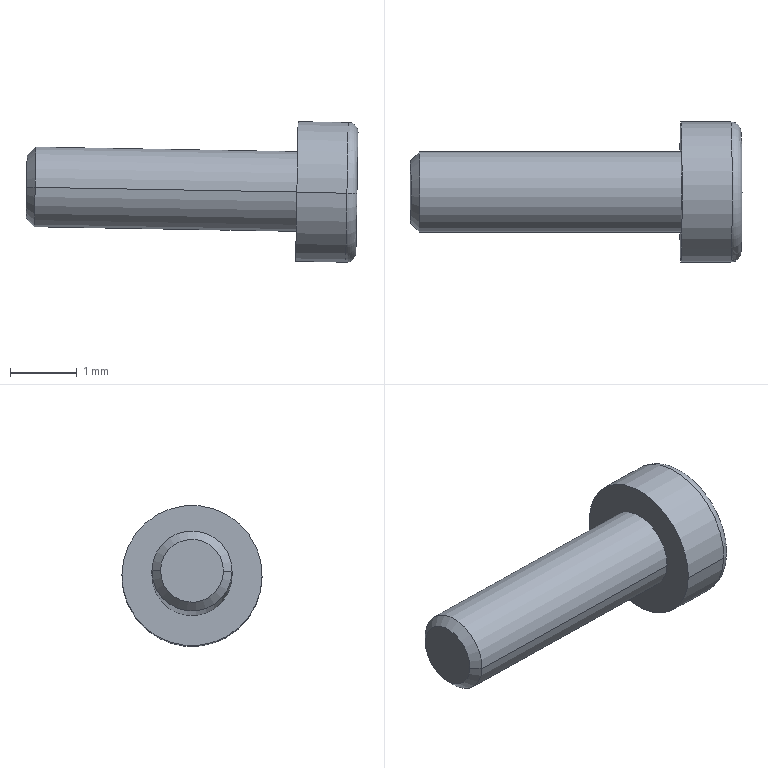Component | SolidWorks | 00-VacuumSuctionCupAssembly-1_05-M4Screw-10 | 1 solid | 18 faces | box 4.97 x 2.1 x 2.11 mm | volume 7 mm3 | plane 10 | cylinder 4 | torus 2 | cone 2 | commonest cylinder face diameters 1.2 x2 2.1 x2
STEP:
#1=COLOUR_RGB('',0.7922,0.8196,0.9333);
#2=FILL_AREA_STYLE_COLOUR('',#1);
#3=FILL_AREA_STYLE('',(#2));
#4=SURFACE_STYLE_FILL_AREA(#3);
#5=SURFACE_SIDE_STYLE('',(#4));
#6=SURFACE_STYLE_USAGE(.BOTH.,#5);
#7=PRESENTATION_STYLE_ASSIGNMENT((#6));
#8=CARTESIAN_POINT('',(2.906,4.646,1.973));
#9=VERTEX_POINT('',#8);
#10=CARTESIAN_POINT('',(2.906,4.563,1.972));
#11=VERTEX_POINT('',#10);
#12=CARTESIAN_POINT('',(2.906,4.604,1.973));
#13=DIRECTION('',(-0.9998,0.,0.01745));
#14=DIRECTION('',(-0.0001976,-0.9999,-0.01132));
#15=AXIS2_PLACEMENT_3D('',#12,#13,#14);
#16=CIRCLE('',#15,0.04134);
#17=EDGE_CURVE('',#9,#11,#16,.T.);
#18=ORIENTED_EDGE('',*,*,#17,.F.);
#19=CARTESIAN_POINT('',(2.912,4.64,1.973));
#20=VERTEX_POINT('',#19);
#21=CARTESIAN_POINT('',(2.906,4.64,1.973));
#22=DIRECTION('',(-0.01745,0.01132,-0.9998));
#23=DIRECTION('',(-0.9998,0.,0.01745));
#24=AXIS2_PLACEMENT_3D('',#21,#22,#23);
#25=CIRCLE('',#24,0.005906);
#26=EDGE_CURVE('',#9,#20,#25,.T.);
#27=ORIENTED_EDGE('',*,*,#26,.T.);
#28=CARTESIAN_POINT('',(2.912,4.569,1.972));
#29=VERTEX_POINT('',#28);
#30=CARTESIAN_POINT('',(2.912,4.604,1.973));
#31=DIRECTION('',(0.9998,-0.,-0.01745));
#32=DIRECTION('',(-0.0001976,-0.9999,-0.01132));
#33=AXIS2_PLACEMENT_3D('',#30,#31,#32);
#34=CIRCLE('',#33,0.03543);
#35=EDGE_CURVE('',#29,#20,#34,.T.);
#36=ORIENTED_EDGE('',*,*,#35,.F.);
#37=CARTESIAN_POINT('',(2.906,4.569,1.972));
#38=DIRECTION('',(0.01745,-0.01132,0.9998));
#39=DIRECTION('',(0.9998,0.,-0.01745));
#40=AXIS2_PLACEMENT_3D('',#37,#38,#39);
#41=CIRCLE('',#40,0.005906);
#42=EDGE_CURVE('',#11,#29,#41,.T.);
#43=ORIENTED_EDGE('',*,*,#42,.F.);
#44=EDGE_LOOP('',(#18,#27,#36,#43));
#45=FACE_OUTER_BOUND('',#44,.T.);
#46=CARTESIAN_POINT('',(2.906,4.604,1.973));
#47=DIRECTION('',(0.9998,-0.,-0.01745));
#48=DIRECTION('',(-0.0001976,-0.9999,-0.01132));
#49=AXIS2_PLACEMENT_3D('',#46,#47,#48);
#50=TOROIDAL_SURFACE('',#49,0.03543,0.005906);
#51=ADVANCED_FACE('',(#45),#50,.T.);
#52=CARTESIAN_POINT('',(2.717,4.623,1.976));
#53=VERTEX_POINT('',#52);
#54=CARTESIAN_POINT('',(2.717,4.586,1.976));
#55=VERTEX_POINT('',#54);
#56=CARTESIAN_POINT('',(2.717,4.604,1.976));
#57=DIRECTION('',(-0.9998,0.,0.01745));
#58=DIRECTION('',(0.0001976,0.9999,0.01132));
#59=AXIS2_PLACEMENT_3D('',#56,#57,#58);
#60=CIRCLE('',#59,0.01855);
#61=EDGE_CURVE('',#53,#55,#60,.T.);
#62=ORIENTED_EDGE('',*,*,#61,.F.);
#63=CARTESIAN_POINT('',(2.722,4.628,1.976));
#64=VERTEX_POINT('',#63);
#65=CARTESIAN_POINT('',(2.717,4.623,1.976));
#66=DIRECTION('',(0.7071,0.7071,-0.004337));
#67=VECTOR('',#66,39.37);
#68=LINE('',#65,#67);
#69=EDGE_CURVE('',#53,#64,#68,.T.);
#70=ORIENTED_EDGE('',*,*,#69,.T.);
#71=CARTESIAN_POINT('',(2.722,4.581,1.976));
#72=VERTEX_POINT('',#71);
#73=CARTESIAN_POINT('',(2.722,4.604,1.976));
#74=DIRECTION('',(0.9998,-0.,-0.01745));
#75=DIRECTION('',(0.0001976,0.9999,0.01132));
#76=AXIS2_PLACEMENT_3D('',#73,#74,#75);
#77=CIRCLE('',#76,0.02362);
#78=EDGE_CURVE('',#72,#64,#77,.T.);
#79=ORIENTED_EDGE('',*,*,#78,.F.);
#80=CARTESIAN_POINT('',(2.717,4.586,1.976));
#81=DIRECTION('',(0.7069,-0.7071,-0.02034));
#82=VECTOR('',#81,39.37);
#83=LINE('',#80,#82);
#84=EDGE_CURVE('',#55,#72,#83,.T.);
#85=ORIENTED_EDGE('',*,*,#84,.F.);
#86=EDGE_LOOP('',(#62,#70,#79,#85));
#87=FACE_OUTER_BOUND('',#86,.T.);
#88=CARTESIAN_POINT('',(2.717,4.604,1.976));
#89=DIRECTION('',(0.9998,-0.,-0.01745));
#90=DIRECTION('',(-0.0001976,-0.9999,-0.01132));
#91=AXIS2_PLACEMENT_3D('',#88,#89,#90);
#92=CONICAL_SURFACE('',#91,0.01855,0.7854);
#93=ADVANCED_FACE('',(#87),#92,.T.);
#94=ORIENTED_EDGE('',*,*,#78,.T.);
#95=CARTESIAN_POINT('',(2.877,4.628,1.974));
#96=VERTEX_POINT('',#95);
#97=CARTESIAN_POINT('',(2.717,4.628,1.976));
#98=DIRECTION('',(0.9998,-0.,-0.01745));
#99=VECTOR('',#98,39.37);
#100=LINE('',#97,#99);
#101=EDGE_CURVE('',#64,#96,#100,.T.);
#102=ORIENTED_EDGE('',*,*,#101,.T.);
#103=CARTESIAN_POINT('',(2.877,4.581,1.973));
#104=VERTEX_POINT('',#103);
#105=CARTESIAN_POINT('',(2.877,4.604,1.973));
#106=DIRECTION('',(-0.9998,0.,0.01745));
#107=DIRECTION('',(0.0001976,0.9999,0.01132));
#108=AXIS2_PLACEMENT_3D('',#105,#106,#107);
#109=CIRCLE('',#108,0.02362);
#110=EDGE_CURVE('',#96,#104,#109,.T.);
#111=ORIENTED_EDGE('',*,*,#110,.T.);
#112=CARTESIAN_POINT('',(2.717,4.581,1.976));
#113=DIRECTION('',(0.9998,-0.,-0.01745));
#114=VECTOR('',#113,39.37);
#115=LINE('',#112,#114);
#116=EDGE_CURVE('',#72,#104,#115,.T.);
#117=ORIENTED_EDGE('',*,*,#116,.F.);
#118=EDGE_LOOP('',(#94,#102,#111,#117));
#119=FACE_OUTER_BOUND('',#118,.T.);
#120=CARTESIAN_POINT('',(2.717,4.604,1.976));
#121=DIRECTION('',(0.9998,-0.,-0.01745));
#122=DIRECTION('',(-0.0001976,-0.9999,-0.01132));
#123=AXIS2_PLACEMENT_3D('',#120,#121,#122);
#124=CYLINDRICAL_SURFACE('',#123,0.02362);
#125=ADVANCED_FACE('',(#119),#124,.T.);
#126=ORIENTED_EDGE('',*,*,#17,.T.);
#127=CARTESIAN_POINT('',(2.877,4.563,1.973));
#128=VERTEX_POINT('',#127);
#129=CARTESIAN_POINT('',(2.912,4.563,1.972));
#130=DIRECTION('',(-0.9998,0.,0.01745));
#131=VECTOR('',#130,39.37);
#132=LINE('',#129,#131);
#133=EDGE_CURVE('',#11,#128,#132,.T.);
#134=ORIENTED_EDGE('',*,*,#133,.T.);
#135=CARTESIAN_POINT('',(2.877,4.646,1.974));
#136=VERTEX_POINT('',#135);
#137=CARTESIAN_POINT('',(2.877,4.604,1.973));
#138=DIRECTION('',(-0.9998,0.,0.01745));
#139=DIRECTION('',(0.0001976,0.9999,0.01132));
#140=AXIS2_PLACEMENT_3D('',#137,#138,#139);
#141=CIRCLE('',#140,0.04134);
#142=EDGE_CURVE('',#136,#128,#141,.T.);
#143=ORIENTED_EDGE('',*,*,#142,.F.);
#144=CARTESIAN_POINT('',(2.912,4.646,1.973));
#145=DIRECTION('',(-0.9998,0.,0.01745));
#146=VECTOR('',#145,39.37);
#147=LINE('',#144,#146);
#148=EDGE_CURVE('',#9,#136,#147,.T.);
#149=ORIENTED_EDGE('',*,*,#148,.F.);
#150=EDGE_LOOP('',(#126,#134,#143,#149));
#151=FACE_OUTER_BOUND('',#150,.T.);
#152=CARTESIAN_POINT('',(2.912,4.604,1.973));
#153=DIRECTION('',(-0.9998,0.,0.01745));
#154=DIRECTION('',(0.0001976,0.9999,0.01132));
#155=AXIS2_PLACEMENT_3D('',#152,#153,#154);
#156=CYLINDRICAL_SURFACE('',#155,0.04134);
#157=ADVANCED_FACE('',(#151),#156,.T.);
#158=ORIENTED_EDGE('',*,*,#142,.T.);
#159=CARTESIAN_POINT('',(2.877,4.604,1.973));
#160=DIRECTION('',(-0.9998,0.,0.01745));
#161=DIRECTION('',(0.0001976,0.9999,0.01132));
#162=AXIS2_PLACEMENT_3D('',#159,#160,#161);
#163=CIRCLE('',#162,0.04134);
#164=EDGE_CURVE('',#128,#136,#163,.T.);
#165=ORIENTED_EDGE('',*,*,#164,.T.);
#166=EDGE_LOOP('',(#158,#165));
#167=FACE_OUTER_BOUND('',#166,.T.);
#168=CARTESIAN_POINT('',(2.877,4.604,1.973));
#169=DIRECTION('',(-0.9998,0.,0.01745));
#170=DIRECTION('',(0.0001976,0.9999,0.01132));
#171=AXIS2_PLACEMENT_3D('',#168,#169,#170);
#172=CIRCLE('',#171,0.02362);
#173=EDGE_CURVE('',#104,#96,#172,.T.);
#174=ORIENTED_EDGE('',*,*,#173,.F.);
#175=ORIENTED_EDGE('',*,*,#110,.F.);
#176=EDGE_LOOP('',(#174,#175));
#177=FACE_BOUND('',#176,.T.);
#178=CARTESIAN_POINT('',(2.877,4.604,1.973));
#179=DIRECTION('',(-0.9998,0.,0.01745));
#180=DIRECTION('',(0.0001976,0.9999,0.01132));
#181=AXIS2_PLACEMENT_3D('',#178,#179,#180);
#182=PLANE('',#181);
#183=ADVANCED_FACE('',(#167,#177),#182,.T.);
#184=ORIENTED_EDGE('',*,*,#133,.F.);
#185=CARTESIAN_POINT('',(2.906,4.604,1.973));
#186=DIRECTION('',(-0.9998,0.,0.01745));
#187=DIRECTION('',(-0.0001976,-0.9999,-0.01132));
#188=AXIS2_PLACEMENT_3D('',#185,#186,#187);
#189=CIRCLE('',#188,0.04134);
#190=EDGE_CURVE('',#11,#9,#189,.T.);
#191=ORIENTED_EDGE('',*,*,#190,.T.);
#192=ORIENTED_EDGE('',*,*,#148,.T.);
#193=ORIENTED_EDGE('',*,*,#164,.F.);
#194=EDGE_LOOP('',(#184,#191,#192,#193));
#195=FACE_OUTER_BOUND('',#194,.T.);
#196=CARTESIAN_POINT('',(2.912,4.604,1.973));
#197=DIRECTION('',(-0.9998,0.,0.01745));
#198=DIRECTION('',(0.0001976,0.9999,0.01132));
#199=AXIS2_PLACEMENT_3D('',#196,#197,#198);
#200=CYLINDRICAL_SURFACE('',#199,0.04134);
#201=ADVANCED_FACE('',(#195),#200,.T.);
#202=ORIENTED_EDGE('',*,*,#35,.T.);
#203=CARTESIAN_POINT('',(2.912,4.604,1.973));
#204=DIRECTION('',(0.9998,-0.,-0.01745));
#205=DIRECTION('',(-0.0001976,-0.9999,-0.01132));
#206=AXIS2_PLACEMENT_3D('',#203,#204,#205);
#207=CIRCLE('',#206,0.03543);
#208=EDGE_CURVE('',#20,#29,#207,.T.);
#209=ORIENTED_EDGE('',*,*,#208,.T.);
#210=EDGE_LOOP('',(#202,#209));
#211=FACE_OUTER_BOUND('',#210,.T.);
#212=CARTESIAN_POINT('',(2.912,4.622,1.983));
#213=VERTEX_POINT('',#212);
#214=CARTESIAN_POINT('',(2.912,4.604,1.993));
#215=VERTEX_POINT('',#214);
#216=CARTESIAN_POINT('',(2.912,4.622,1.983));
#217=DIRECTION('',(0.008555,-0.8716,0.4901));
#218=VECTOR('',#217,39.37);
#219=LINE('',#216,#218);
#220=EDGE_CURVE('',#213,#215,#219,.T.);
#221=ORIENTED_EDGE('',*,*,#220,.F.);
#222=CARTESIAN_POINT('',(2.912,4.622,1.963));
#223=VERTEX_POINT('',#222);
#224=CARTESIAN_POINT('',(2.912,4.622,1.963));
#225=DIRECTION('',(0.01745,-0.01132,0.9998));
#226=VECTOR('',#225,39.37);
#227=LINE('',#224,#226);
#228=EDGE_CURVE('',#223,#213,#227,.T.);
#229=ORIENTED_EDGE('',*,*,#228,.F.);
#230=CARTESIAN_POINT('',(2.912,4.605,1.952));
#231=VERTEX_POINT('',#230);
#232=CARTESIAN_POINT('',(2.912,4.605,1.952));
#233=DIRECTION('',(0.008897,0.8603,0.5097));
#234=VECTOR('',#233,39.37);
#235=LINE('',#232,#234);
#236=EDGE_CURVE('',#231,#223,#235,.T.);
#237=ORIENTED_EDGE('',*,*,#236,.F.);
#238=CARTESIAN_POINT('',(2.912,4.587,1.962));
#239=VERTEX_POINT('',#238);
#240=CARTESIAN_POINT('',(2.912,4.587,1.962));
#241=DIRECTION('',(-0.008555,0.8716,-0.4901));
#242=VECTOR('',#241,39.37);
#243=LINE('',#240,#242);
#244=EDGE_CURVE('',#239,#231,#243,.T.);
#245=ORIENTED_EDGE('',*,*,#244,.F.);
#246=CARTESIAN_POINT('',(2.912,4.586,1.983));
#247=VERTEX_POINT('',#246);
#248=CARTESIAN_POINT('',(2.912,4.586,1.983));
#249=DIRECTION('',(-0.01745,0.01132,-0.9998));
#250=VECTOR('',#249,39.37);
#251=LINE('',#248,#250);
#252=EDGE_CURVE('',#247,#239,#251,.T.);
#253=ORIENTED_EDGE('',*,*,#252,.F.);
#254=CARTESIAN_POINT('',(2.912,4.604,1.993));
#255=DIRECTION('',(-0.008897,-0.8603,-0.5097));
#256=VECTOR('',#255,39.37);
#257=LINE('',#254,#256);
#258=EDGE_CURVE('',#215,#247,#257,.T.);
#259=ORIENTED_EDGE('',*,*,#258,.F.);
#260=EDGE_LOOP('',(#221,#229,#237,#245,#253,#259));
#261=FACE_BOUND('',#260,.T.);
#262=CARTESIAN_POINT('',(2.911,4.605,1.931));
#263=DIRECTION('',(0.9998,-0.,-0.01745));
#264=DIRECTION('',(-0.0001976,-0.9999,-0.01132));
#265=AXIS2_PLACEMENT_3D('',#262,#263,#264);
#266=PLANE('',#265);
#267=ADVANCED_FACE('',(#211,#261),#266,.T.);
#268=ORIENTED_EDGE('',*,*,#101,.F.);
#269=CARTESIAN_POINT('',(2.722,4.604,1.976));
#270=DIRECTION('',(0.9998,-0.,-0.01745));
#271=DIRECTION('',(0.0001976,0.9999,0.01132));
#272=AXIS2_PLACEMENT_3D('',#269,#270,#271);
#273=CIRCLE('',#272,0.02362);
#274=EDGE_CURVE('',#64,#72,#273,.T.);
#275=ORIENTED_EDGE('',*,*,#274,.T.);
#276=ORIENTED_EDGE('',*,*,#116,.T.);
#277=ORIENTED_EDGE('',*,*,#173,.T.);
#278=EDGE_LOOP('',(#268,#275,#276,#277));
#279=FACE_OUTER_BOUND('',#278,.T.);
#280=CARTESIAN_POINT('',(2.717,4.604,1.976));
#281=DIRECTION('',(0.9998,-0.,-0.01745));
#282=DIRECTION('',(-0.0001976,-0.9999,-0.01132));
#283=AXIS2_PLACEMENT_3D('',#280,#281,#282);
#284=CYLINDRICAL_SURFACE('',#283,0.02362);
#285=ADVANCED_FACE('',(#279),#284,.T.);
#286=CARTESIAN_POINT('',(2.717,4.604,1.976));
#287=DIRECTION('',(-0.9998,0.,0.01745));
#288=DIRECTION('',(0.0001976,0.9999,0.01132));
#289=AXIS2_PLACEMENT_3D('',#286,#287,#288);
#290=CIRCLE('',#289,0.01855);
#291=EDGE_CURVE('',#55,#53,#290,.T.);
#292=ORIENTED_EDGE('',*,*,#291,.T.);
#293=ORIENTED_EDGE('',*,*,#61,.T.);
#294=EDGE_LOOP('',(#292,#293));
#295=FACE_OUTER_BOUND('',#294,.T.);
#296=CARTESIAN_POINT('',(2.717,4.604,1.976));
#297=DIRECTION('',(-0.9998,0.,0.01745));
#298=DIRECTION('',(0.0001976,0.9999,0.01132));
#299=AXIS2_PLACEMENT_3D('',#296,#297,#298);
#300=PLANE('',#299);
#301=ADVANCED_FACE('',(#295),#300,.T.);
#302=ORIENTED_EDGE('',*,*,#220,.T.);
#303=CARTESIAN_POINT('',(2.889,4.604,1.994));
#304=VERTEX_POINT('',#303);
#305=CARTESIAN_POINT('',(2.889,4.604,1.994));
#306=DIRECTION('',(0.9998,-0.,-0.01745));
#307=VECTOR('',#306,39.37);
#308=LINE('',#305,#307);
#309=EDGE_CURVE('',#304,#215,#308,.T.);
#310=ORIENTED_EDGE('',*,*,#309,.F.);
#311=CARTESIAN_POINT('',(2.889,4.622,1.984));
#312=VERTEX_POINT('',#311);
#313=CARTESIAN_POINT('',(2.889,4.622,1.984));
#314=DIRECTION('',(0.008555,-0.8716,0.4901));
#315=VECTOR('',#314,39.37);
#316=LINE('',#313,#315);
#317=EDGE_CURVE('',#312,#304,#316,.T.);
#318=ORIENTED_EDGE('',*,*,#317,.F.);
#319=CARTESIAN_POINT('',(2.889,4.622,1.984));
#320=DIRECTION('',(0.9998,-0.,-0.01745));
#321=VECTOR('',#320,39.37);
#322=LINE('',#319,#321);
#323=EDGE_CURVE('',#312,#213,#322,.T.);
#324=ORIENTED_EDGE('',*,*,#323,.T.);
#325=EDGE_LOOP('',(#302,#310,#318,#324));
#326=FACE_OUTER_BOUND('',#325,.T.);
#327=CARTESIAN_POINT('',(2.889,4.622,1.984));
#328=DIRECTION('',(0.01521,0.4902,0.8715));
#329=DIRECTION('',(-0.008555,0.8716,-0.4901));
#330=AXIS2_PLACEMENT_3D('',#327,#328,#329);
#331=PLANE('',#330);
#332=ADVANCED_FACE('',(#326),#331,.F.);
#333=ORIENTED_EDGE('',*,*,#228,.T.);
#334=ORIENTED_EDGE('',*,*,#323,.F.);
#335=CARTESIAN_POINT('',(2.888,4.622,1.963));
#336=VERTEX_POINT('',#335);
#337=CARTESIAN_POINT('',(2.888,4.622,1.963));
#338=DIRECTION('',(0.01745,-0.01132,0.9998));
#339=VECTOR('',#338,39.37);
#340=LINE('',#337,#339);
#341=EDGE_CURVE('',#336,#312,#340,.T.);
#342=ORIENTED_EDGE('',*,*,#341,.F.);
#343=CARTESIAN_POINT('',(2.888,4.622,1.963));
#344=DIRECTION('',(0.9998,-0.,-0.01745));
#345=VECTOR('',#344,39.37);
#346=LINE('',#343,#345);
#347=EDGE_CURVE('',#336,#223,#346,.T.);
#348=ORIENTED_EDGE('',*,*,#347,.T.);
#349=EDGE_LOOP('',(#333,#334,#342,#348));
#350=FACE_OUTER_BOUND('',#349,.T.);
#351=CARTESIAN_POINT('',(2.888,4.622,1.963));
#352=DIRECTION('',(0.0001976,0.9999,0.01132));
#353=DIRECTION('',(0.9998,-0.,-0.01745));
#354=AXIS2_PLACEMENT_3D('',#351,#352,#353);
#355=PLANE('',#354);
#356=ADVANCED_FACE('',(#350),#355,.F.);
#357=ORIENTED_EDGE('',*,*,#236,.T.);
#358=ORIENTED_EDGE('',*,*,#347,.F.);
#359=CARTESIAN_POINT('',(2.888,4.605,1.953));
#360=VERTEX_POINT('',#359);
#361=CARTESIAN_POINT('',(2.888,4.605,1.953));
#362=DIRECTION('',(0.008897,0.8603,0.5097));
#363=VECTOR('',#362,39.37);
#364=LINE('',#361,#363);
#365=EDGE_CURVE('',#360,#336,#364,.T.);
#366=ORIENTED_EDGE('',*,*,#365,.F.);
#367=CARTESIAN_POINT('',(2.888,4.605,1.953));
#368=DIRECTION('',(0.9998,-0.,-0.01745));
#369=VECTOR('',#368,39.37);
#370=LINE('',#367,#369);
#371=EDGE_CURVE('',#360,#231,#370,.T.);
#372=ORIENTED_EDGE('',*,*,#371,.T.);
#373=EDGE_LOOP('',(#357,#358,#366,#372));
#374=FACE_OUTER_BOUND('',#373,.T.);
#375=CARTESIAN_POINT('',(2.888,4.605,1.953));
#376=DIRECTION('',(-0.01501,0.5098,-0.8602));
#377=DIRECTION('',(-0.008897,-0.8603,-0.5097));
#378=AXIS2_PLACEMENT_3D('',#375,#376,#377);
#379=PLANE('',#378);
#380=ADVANCED_FACE('',(#374),#379,.F.);
#381=ORIENTED_EDGE('',*,*,#244,.T.);
#382=ORIENTED_EDGE('',*,*,#371,.F.);
#383=CARTESIAN_POINT('',(2.888,4.587,1.963));
#384=VERTEX_POINT('',#383);
#385=CARTESIAN_POINT('',(2.888,4.587,1.963));
#386=DIRECTION('',(-0.008555,0.8716,-0.4901));
#387=VECTOR('',#386,39.37);
#388=LINE('',#385,#387);
#389=EDGE_CURVE('',#384,#360,#388,.T.);
#390=ORIENTED_EDGE('',*,*,#389,.F.);
#391=CARTESIAN_POINT('',(2.888,4.587,1.963));
#392=DIRECTION('',(0.9998,-0.,-0.01745));
#393=VECTOR('',#392,39.37);
#394=LINE('',#391,#393);
#395=EDGE_CURVE('',#384,#239,#394,.T.);
#396=ORIENTED_EDGE('',*,*,#395,.T.);
#397=EDGE_LOOP('',(#381,#382,#390,#396));
#398=FACE_OUTER_BOUND('',#397,.T.);
#399=CARTESIAN_POINT('',(2.888,4.587,1.963));
#400=DIRECTION('',(-0.01521,-0.4902,-0.8715));
#401=DIRECTION('',(0.008555,-0.8716,0.4901));
#402=AXIS2_PLACEMENT_3D('',#399,#400,#401);
#403=PLANE('',#402);
#404=ADVANCED_FACE('',(#398),#403,.F.);
#405=ORIENTED_EDGE('',*,*,#252,.T.);
#406=ORIENTED_EDGE('',*,*,#395,.F.);
#407=CARTESIAN_POINT('',(2.889,4.586,1.983));
#408=VERTEX_POINT('',#407);
#409=CARTESIAN_POINT('',(2.889,4.586,1.983));
#410=DIRECTION('',(-0.01745,0.01132,-0.9998));
#411=VECTOR('',#410,39.37);
#412=LINE('',#409,#411);
#413=EDGE_CURVE('',#408,#384,#412,.T.);
#414=ORIENTED_EDGE('',*,*,#413,.F.);
#415=CARTESIAN_POINT('',(2.889,4.586,1.983));
#416=DIRECTION('',(0.9998,-0.,-0.01745));
#417=VECTOR('',#416,39.37);
#418=LINE('',#415,#417);
#419=EDGE_CURVE('',#408,#247,#418,.T.);
#420=ORIENTED_EDGE('',*,*,#419,.T.);
#421=EDGE_LOOP('',(#405,#406,#414,#420));
#422=FACE_OUTER_BOUND('',#421,.T.);
#423=CARTESIAN_POINT('',(2.889,4.586,1.983));
#424=DIRECTION('',(-0.0001976,-0.9999,-0.01132));
#425=DIRECTION('',(-0.9998,0.,0.01745));
#426=AXIS2_PLACEMENT_3D('',#423,#424,#425);
#427=PLANE('',#426);
#428=ADVANCED_FACE('',(#422),#427,.F.);
#429=ORIENTED_EDGE('',*,*,#258,.T.);
#430=ORIENTED_EDGE('',*,*,#419,.F.);
#431=CARTESIAN_POINT('',(2.889,4.604,1.994));
#432=DIRECTION('',(-0.008897,-0.8603,-0.5097));
#433=VECTOR('',#432,39.37);
#434=LINE('',#431,#433);
#435=EDGE_CURVE('',#304,#408,#434,.T.);
#436=ORIENTED_EDGE('',*,*,#435,.F.);
#437=ORIENTED_EDGE('',*,*,#309,.T.);
#438=EDGE_LOOP('',(#429,#430,#436,#437));
#439=FACE_OUTER_BOUND('',#438,.T.);
#440=CARTESIAN_POINT('',(2.889,4.604,1.994));
#441=DIRECTION('',(0.01501,-0.5098,0.8602));
#442=DIRECTION('',(0.008897,0.8603,0.5097));
#443=AXIS2_PLACEMENT_3D('',#440,#441,#442);
#444=PLANE('',#443);
#445=ADVANCED_FACE('',(#439),#444,.F.);
#446=ORIENTED_EDGE('',*,*,#317,.T.);
#447=ORIENTED_EDGE('',*,*,#435,.T.);
#448=ORIENTED_EDGE('',*,*,#413,.T.);
#449=ORIENTED_EDGE('',*,*,#389,.T.);
#450=ORIENTED_EDGE('',*,*,#365,.T.);
#451=ORIENTED_EDGE('',*,*,#341,.T.);
#452=EDGE_LOOP('',(#446,#447,#448,#449,#450,#451));
#453=FACE_OUTER_BOUND('',#452,.T.);
#454=CARTESIAN_POINT('',(2.888,4.604,1.973));
#455=DIRECTION('',(0.9998,-0.,-0.01745));
#456=DIRECTION('',(-0.0001976,-0.9999,-0.01132));
#457=AXIS2_PLACEMENT_3D('',#454,#455,#456);
#458=PLANE('',#457);
#459=ADVANCED_FACE('',(#453),#458,.T.);
#460=ORIENTED_EDGE('',*,*,#69,.F.);
#461=ORIENTED_EDGE('',*,*,#291,.F.);
#462=ORIENTED_EDGE('',*,*,#84,.T.);
#463=ORIENTED_EDGE('',*,*,#274,.F.);
#464=EDGE_LOOP('',(#460,#461,#462,#463));
#465=FACE_OUTER_BOUND('',#464,.T.);
#466=CARTESIAN_POINT('',(2.717,4.604,1.976));
#467=DIRECTION('',(0.9998,-0.,-0.01745));
#468=DIRECTION('',(-0.0001976,-0.9999,-0.01132));
#469=AXIS2_PLACEMENT_3D('',#466,#467,#468);
#470=CONICAL_SURFACE('',#469,0.01855,0.7854);
#471=ADVANCED_FACE('',(#465),#470,.T.);
#472=ORIENTED_EDGE('',*,*,#26,.F.);
#473=ORIENTED_EDGE('',*,*,#190,.F.);
#474=ORIENTED_EDGE('',*,*,#42,.T.);
#475=ORIENTED_EDGE('',*,*,#208,.F.);
#476=EDGE_LOOP('',(#472,#473,#474,#475));
#477=FACE_OUTER_BOUND('',#476,.T.);
#478=CARTESIAN_POINT('',(2.906,4.604,1.973));
#479=DIRECTION('',(0.9998,-0.,-0.01745));
#480=DIRECTION('',(-0.0001976,-0.9999,-0.01132));
#481=AXIS2_PLACEMENT_3D('',#478,#479,#480);
#482=TOROIDAL_SURFACE('',#481,0.03543,0.005906);
#483=ADVANCED_FACE('',(#477),#482,.T.);
#484=CLOSED_SHELL('',(#51,#93,#125,#157,#183,#201,#267,#285,#301,#332,#356,#380,#404,#428,#445,#459,#471,#483));
#485=MANIFOLD_SOLID_BREP('',#484);
#486=STYLED_ITEM('',(#7),#485);
#487=(LENGTH_UNIT()NAMED_UNIT(*)SI_UNIT($,.METRE.));
#488=LENGTH_MEASURE_WITH_UNIT(LENGTH_MEASURE(0.0254),#487);
#489=DIMENSIONAL_EXPONENTS(1.,0.,0.,0.,0.,0.,0.);
#490=(CONVERSION_BASED_UNIT('',#488)LENGTH_UNIT()NAMED_UNIT(#489));
#491=UNCERTAINTY_MEASURE_WITH_UNIT(LENGTH_MEASURE(0.00001),#490,'','');
#492=(NAMED_UNIT(*)PLANE_ANGLE_UNIT()SI_UNIT($,.RADIAN.));
#493=(NAMED_UNIT(*)SI_UNIT($,.STERADIAN.)SOLID_ANGLE_UNIT());
#494=(GEOMETRIC_REPRESENTATION_CONTEXT(3)GLOBAL_UNCERTAINTY_ASSIGNED_CONTEXT((#491))GLOBAL_UNIT_ASSIGNED_CONTEXT((#490,#492,#493))REPRESENTATION_CONTEXT('',''));
#495=MECHANICAL_DESIGN_GEOMETRIC_PRESENTATION_REPRESENTATION('',(#486),#494);
#496=CARTESIAN_POINT('',(0.,0.,0.));
#497=DIRECTION('',(0.,0.,1.));
#498=DIRECTION('',(1.,0.,0.));
#499=AXIS2_PLACEMENT_3D('',#496,#497,#498);
#500=(LENGTH_UNIT()NAMED_UNIT(*)SI_UNIT($,.METRE.));
#501=LENGTH_MEASURE_WITH_UNIT(LENGTH_MEASURE(0.0254),#500);
#502=DIMENSIONAL_EXPONENTS(1.,0.,0.,0.,0.,0.,0.);
#503=(CONVERSION_BASED_UNIT('',#501)LENGTH_UNIT()NAMED_UNIT(#502));
#504=UNCERTAINTY_MEASURE_WITH_UNIT(LENGTH_MEASURE(0.00001),#503,'','');
#505=(NAMED_UNIT(*)PLANE_ANGLE_UNIT()SI_UNIT($,.RADIAN.));
#506=(NAMED_UNIT(*)SI_UNIT($,.STERADIAN.)SOLID_ANGLE_UNIT());
#507=(GEOMETRIC_REPRESENTATION_CONTEXT(3)GLOBAL_UNCERTAINTY_ASSIGNED_CONTEXT((#504))GLOBAL_UNIT_ASSIGNED_CONTEXT((#503,#505,#506))REPRESENTATION_CONTEXT('',''));
#508=ADVANCED_BREP_SHAPE_REPRESENTATION('',(#485,#499),#507);
#509=PRESENTATION_LAYER_ASSIGNMENT('','',(#486));